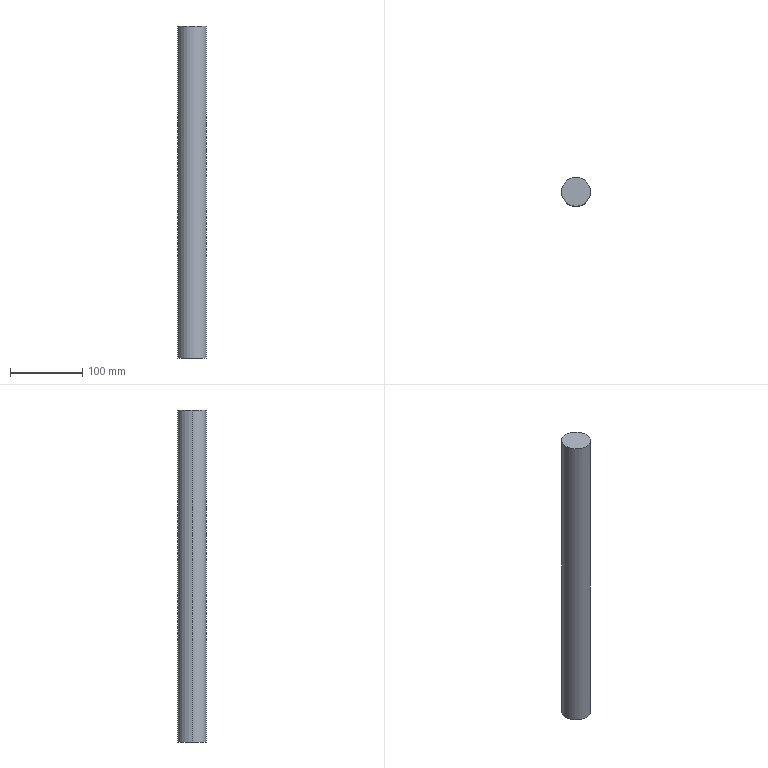Component | SolidWorks | 40Axis-4 | 1 solid | 12 faces | box 40 x 40 x 460 mm | volume 576569 mm3 | cylinder 6 | cone 4 | plane 2 | commonest cylinder face diameters 6.8 x4 40 x2 | material 45#
build123d program:
from build123d import *

# Parameters (mm, degrees)
SKETCH1_R             = 20
BOSS_EXTRUDE1_DEPTH   = 230
M8_TAPPED_HOLE1_D     = 6.8
M8_TAPPED_HOLE1_DEPTH = 19.75
M8_TAPPED_HOLE1_TIP   = 2.043


with BuildPart() as part:
    # Sketch1 → Boss-Extrude1 (new, symmetric)
    with BuildSketch(Plane.XY):
        Circle(SKETCH1_R)
    extrude(amount=BOSS_EXTRUDE1_DEPTH, both=True)

    # M8 Tapped Hole1
    with Locations(Plane(origin=(-10, 0, -230), x_dir=(-1, 0, 0), z_dir=(0, 0, -1))):
        with Locations((0, 0), (-20, 0)):
            Hole(M8_TAPPED_HOLE1_D / 2, depth=M8_TAPPED_HOLE1_DEPTH)
            with Locations((0, 0, -(M8_TAPPED_HOLE1_DEPTH + M8_TAPPED_HOLE1_TIP / 2))):  # 118° drill point
                Cone(0, M8_TAPPED_HOLE1_D / 2, M8_TAPPED_HOLE1_TIP, mode=Mode.SUBTRACT)


solid = part.part

# Placed as in the assembly
solid = solid.moved(Location((-218.215, 103.083, -950.957), (0, 0, 0)))
STEP:
#1=COLOUR_RGB('',0.7922,0.8196,0.9333);
#2=FILL_AREA_STYLE_COLOUR('',#1);
#3=FILL_AREA_STYLE('',(#2));
#4=SURFACE_STYLE_FILL_AREA(#3);
#5=SURFACE_SIDE_STYLE('',(#4));
#6=SURFACE_STYLE_USAGE(.BOTH.,#5);
#7=PRESENTATION_STYLE_ASSIGNMENT((#6));
#8=CARTESIAN_POINT('',(-8.331,4.058,-45.717));
#9=VERTEX_POINT('',#8);
#10=CARTESIAN_POINT('',(-8.064,4.058,-45.717));
#11=VERTEX_POINT('',#10);
#12=CARTESIAN_POINT('',(-8.197,4.058,-45.717));
#13=DIRECTION('',(0.,-0.,-1.));
#14=DIRECTION('',(1.,0.,0.));
#15=AXIS2_PLACEMENT_3D('',#12,#13,#14);
#16=CIRCLE('',#15,0.1339);
#17=EDGE_CURVE('',#9,#11,#16,.T.);
#18=ORIENTED_EDGE('',*,*,#17,.F.);
#19=CARTESIAN_POINT('',(-8.331,4.058,-46.494));
#20=VERTEX_POINT('',#19);
#21=CARTESIAN_POINT('',(-8.331,4.058,-46.494));
#22=DIRECTION('',(0.,-0.,-1.));
#23=VECTOR('',#22,39.37);
#24=LINE('',#21,#23);
#25=EDGE_CURVE('',#9,#20,#24,.T.);
#26=ORIENTED_EDGE('',*,*,#25,.T.);
#27=CARTESIAN_POINT('',(-8.064,4.058,-46.494));
#28=VERTEX_POINT('',#27);
#29=CARTESIAN_POINT('',(-8.197,4.058,-46.494));
#30=DIRECTION('',(0.,-0.,-1.));
#31=DIRECTION('',(1.,0.,0.));
#32=AXIS2_PLACEMENT_3D('',#29,#30,#31);
#33=CIRCLE('',#32,0.1339);
#34=EDGE_CURVE('',#20,#28,#33,.T.);
#35=ORIENTED_EDGE('',*,*,#34,.T.);
#36=CARTESIAN_POINT('',(-8.064,4.058,-46.494));
#37=DIRECTION('',(0.,-0.,-1.));
#38=VECTOR('',#37,39.37);
#39=LINE('',#36,#38);
#40=EDGE_CURVE('',#11,#28,#39,.T.);
#41=ORIENTED_EDGE('',*,*,#40,.F.);
#42=EDGE_LOOP('',(#18,#26,#35,#41));
#43=FACE_OUTER_BOUND('',#42,.T.);
#44=CARTESIAN_POINT('',(-8.197,4.058,-46.494));
#45=DIRECTION('',(0.,-0.,-1.));
#46=DIRECTION('',(1.,0.,0.));
#47=AXIS2_PLACEMENT_3D('',#44,#45,#46);
#48=CYLINDRICAL_SURFACE('',#47,0.1339);
#49=ADVANCED_FACE('',(#43),#48,.F.);
#50=CARTESIAN_POINT('',(-8.197,4.058,-45.636));
#51=VERTEX_POINT('',#50);
#52=CARTESIAN_POINT('',(-8.064,4.058,-45.717));
#53=DIRECTION('',(0.8572,0.,-0.515));
#54=VECTOR('',#53,39.37);
#55=LINE('',#52,#54);
#56=EDGE_CURVE('',#51,#11,#55,.T.);
#57=ORIENTED_EDGE('',*,*,#56,.F.);
#58=CARTESIAN_POINT('',(-8.331,4.058,-45.717));
#59=DIRECTION('',(-0.8572,-0.,-0.515));
#60=VECTOR('',#59,39.37);
#61=LINE('',#58,#60);
#62=EDGE_CURVE('',#51,#9,#61,.T.);
#63=ORIENTED_EDGE('',*,*,#62,.T.);
#64=ORIENTED_EDGE('',*,*,#17,.T.);
#65=EDGE_LOOP('',(#57,#63,#64));
#66=FACE_OUTER_BOUND('',#65,.T.);
#67=CARTESIAN_POINT('',(-8.197,4.058,-45.717));
#68=DIRECTION('',(0.,-0.,-1.));
#69=DIRECTION('',(1.,0.,0.));
#70=AXIS2_PLACEMENT_3D('',#67,#68,#69);
#71=CONICAL_SURFACE('',#70,0.1339,1.03);
#72=ADVANCED_FACE('',(#66),#71,.F.);
#73=CARTESIAN_POINT('',(-9.119,4.058,-45.717));
#74=VERTEX_POINT('',#73);
#75=CARTESIAN_POINT('',(-8.851,4.058,-45.717));
#76=VERTEX_POINT('',#75);
#77=CARTESIAN_POINT('',(-8.985,4.058,-45.717));
#78=DIRECTION('',(0.,-0.,-1.));
#79=DIRECTION('',(1.,0.,0.));
#80=AXIS2_PLACEMENT_3D('',#77,#78,#79);
#81=CIRCLE('',#80,0.1339);
#82=EDGE_CURVE('',#74,#76,#81,.T.);
#83=ORIENTED_EDGE('',*,*,#82,.F.);
#84=CARTESIAN_POINT('',(-9.119,4.058,-46.494));
#85=VERTEX_POINT('',#84);
#86=CARTESIAN_POINT('',(-9.119,4.058,-46.494));
#87=DIRECTION('',(0.,-0.,-1.));
#88=VECTOR('',#87,39.37);
#89=LINE('',#86,#88);
#90=EDGE_CURVE('',#74,#85,#89,.T.);
#91=ORIENTED_EDGE('',*,*,#90,.T.);
#92=CARTESIAN_POINT('',(-8.851,4.058,-46.494));
#93=VERTEX_POINT('',#92);
#94=CARTESIAN_POINT('',(-8.985,4.058,-46.494));
#95=DIRECTION('',(0.,-0.,-1.));
#96=DIRECTION('',(1.,0.,0.));
#97=AXIS2_PLACEMENT_3D('',#94,#95,#96);
#98=CIRCLE('',#97,0.1339);
#99=EDGE_CURVE('',#85,#93,#98,.T.);
#100=ORIENTED_EDGE('',*,*,#99,.T.);
#101=CARTESIAN_POINT('',(-8.851,4.058,-46.494));
#102=DIRECTION('',(0.,-0.,-1.));
#103=VECTOR('',#102,39.37);
#104=LINE('',#101,#103);
#105=EDGE_CURVE('',#76,#93,#104,.T.);
#106=ORIENTED_EDGE('',*,*,#105,.F.);
#107=EDGE_LOOP('',(#83,#91,#100,#106));
#108=FACE_OUTER_BOUND('',#107,.T.);
#109=CARTESIAN_POINT('',(-8.985,4.058,-46.494));
#110=DIRECTION('',(0.,-0.,-1.));
#111=DIRECTION('',(1.,0.,0.));
#112=AXIS2_PLACEMENT_3D('',#109,#110,#111);
#113=CYLINDRICAL_SURFACE('',#112,0.1339);
#114=ADVANCED_FACE('',(#108),#113,.F.);
#115=CARTESIAN_POINT('',(-8.985,4.058,-45.636));
#116=VERTEX_POINT('',#115);
#117=CARTESIAN_POINT('',(-8.851,4.058,-45.717));
#118=DIRECTION('',(0.8572,0.,-0.515));
#119=VECTOR('',#118,39.37);
#120=LINE('',#117,#119);
#121=EDGE_CURVE('',#116,#76,#120,.T.);
#122=ORIENTED_EDGE('',*,*,#121,.F.);
#123=CARTESIAN_POINT('',(-9.119,4.058,-45.717));
#124=DIRECTION('',(-0.8572,-0.,-0.515));
#125=VECTOR('',#124,39.37);
#126=LINE('',#123,#125);
#127=EDGE_CURVE('',#116,#74,#126,.T.);
#128=ORIENTED_EDGE('',*,*,#127,.T.);
#129=ORIENTED_EDGE('',*,*,#82,.T.);
#130=EDGE_LOOP('',(#122,#128,#129));
#131=FACE_OUTER_BOUND('',#130,.T.);
#132=CARTESIAN_POINT('',(-8.985,4.058,-45.717));
#133=DIRECTION('',(0.,-0.,-1.));
#134=DIRECTION('',(1.,0.,0.));
#135=AXIS2_PLACEMENT_3D('',#132,#133,#134);
#136=CONICAL_SURFACE('',#135,0.1339,1.03);
#137=ADVANCED_FACE('',(#131),#136,.F.);
#138=CARTESIAN_POINT('',(-9.379,4.058,-28.384));
#139=VERTEX_POINT('',#138);
#140=CARTESIAN_POINT('',(-7.804,4.058,-28.384));
#141=VERTEX_POINT('',#140);
#142=CARTESIAN_POINT('',(-8.591,4.058,-28.384));
#143=DIRECTION('',(-0.,0.,1.));
#144=DIRECTION('',(-1.,-0.,0.));
#145=AXIS2_PLACEMENT_3D('',#142,#143,#144);
#146=CIRCLE('',#145,0.7874);
#147=EDGE_CURVE('',#139,#141,#146,.T.);
#148=ORIENTED_EDGE('',*,*,#147,.F.);
#149=CARTESIAN_POINT('',(-9.379,4.058,-46.494));
#150=VERTEX_POINT('',#149);
#151=CARTESIAN_POINT('',(-9.379,4.058,-28.384));
#152=DIRECTION('',(0.,-0.,-1.));
#153=VECTOR('',#152,39.37);
#154=LINE('',#151,#153);
#155=EDGE_CURVE('',#139,#150,#154,.T.);
#156=ORIENTED_EDGE('',*,*,#155,.T.);
#157=CARTESIAN_POINT('',(-7.804,4.058,-46.494));
#158=VERTEX_POINT('',#157);
#159=CARTESIAN_POINT('',(-8.591,4.058,-46.494));
#160=DIRECTION('',(-0.,0.,1.));
#161=DIRECTION('',(-1.,-0.,0.));
#162=AXIS2_PLACEMENT_3D('',#159,#160,#161);
#163=CIRCLE('',#162,0.7874);
#164=EDGE_CURVE('',#150,#158,#163,.T.);
#165=ORIENTED_EDGE('',*,*,#164,.T.);
#166=CARTESIAN_POINT('',(-7.804,4.058,-28.384));
#167=DIRECTION('',(0.,-0.,-1.));
#168=VECTOR('',#167,39.37);
#169=LINE('',#166,#168);
#170=EDGE_CURVE('',#141,#158,#169,.T.);
#171=ORIENTED_EDGE('',*,*,#170,.F.);
#172=EDGE_LOOP('',(#148,#156,#165,#171));
#173=FACE_OUTER_BOUND('',#172,.T.);
#174=CARTESIAN_POINT('',(-8.591,4.058,-28.384));
#175=DIRECTION('',(0.,-0.,-1.));
#176=DIRECTION('',(1.,0.,0.));
#177=AXIS2_PLACEMENT_3D('',#174,#175,#176);
#178=CYLINDRICAL_SURFACE('',#177,0.7874);
#179=ADVANCED_FACE('',(#173),#178,.T.);
#180=ORIENTED_EDGE('',*,*,#155,.F.);
#181=CARTESIAN_POINT('',(-8.591,4.058,-28.384));
#182=DIRECTION('',(-0.,0.,1.));
#183=DIRECTION('',(-1.,-0.,0.));
#184=AXIS2_PLACEMENT_3D('',#181,#182,#183);
#185=CIRCLE('',#184,0.7874);
#186=EDGE_CURVE('',#141,#139,#185,.T.);
#187=ORIENTED_EDGE('',*,*,#186,.F.);
#188=ORIENTED_EDGE('',*,*,#170,.T.);
#189=CARTESIAN_POINT('',(-8.591,4.058,-46.494));
#190=DIRECTION('',(-0.,0.,1.));
#191=DIRECTION('',(-1.,-0.,0.));
#192=AXIS2_PLACEMENT_3D('',#189,#190,#191);
#193=CIRCLE('',#192,0.7874);
#194=EDGE_CURVE('',#158,#150,#193,.T.);
#195=ORIENTED_EDGE('',*,*,#194,.T.);
#196=EDGE_LOOP('',(#180,#187,#188,#195));
#197=FACE_OUTER_BOUND('',#196,.T.);
#198=CARTESIAN_POINT('',(-8.591,4.058,-28.384));
#199=DIRECTION('',(0.,-0.,-1.));
#200=DIRECTION('',(1.,0.,0.));
#201=AXIS2_PLACEMENT_3D('',#198,#199,#200);
#202=CYLINDRICAL_SURFACE('',#201,0.7874);
#203=ADVANCED_FACE('',(#197),#202,.T.);
#204=ORIENTED_EDGE('',*,*,#186,.T.);
#205=ORIENTED_EDGE('',*,*,#147,.T.);
#206=EDGE_LOOP('',(#204,#205));
#207=FACE_OUTER_BOUND('',#206,.T.);
#208=CARTESIAN_POINT('',(-8.591,4.058,-28.384));
#209=DIRECTION('',(-0.,0.,1.));
#210=DIRECTION('',(-1.,-0.,-0.));
#211=AXIS2_PLACEMENT_3D('',#208,#209,#210);
#212=PLANE('',#211);
#213=ADVANCED_FACE('',(#207),#212,.T.);
#214=CARTESIAN_POINT('',(-8.197,4.058,-46.494));
#215=DIRECTION('',(0.,-0.,-1.));
#216=DIRECTION('',(1.,0.,0.));
#217=AXIS2_PLACEMENT_3D('',#214,#215,#216);
#218=CIRCLE('',#217,0.1339);
#219=EDGE_CURVE('',#28,#20,#218,.T.);
#220=ORIENTED_EDGE('',*,*,#219,.F.);
#221=ORIENTED_EDGE('',*,*,#34,.F.);
#222=EDGE_LOOP('',(#220,#221));
#223=FACE_BOUND('',#222,.T.);
#224=CARTESIAN_POINT('',(-8.985,4.058,-46.494));
#225=DIRECTION('',(0.,-0.,-1.));
#226=DIRECTION('',(1.,0.,0.));
#227=AXIS2_PLACEMENT_3D('',#224,#225,#226);
#228=CIRCLE('',#227,0.1339);
#229=EDGE_CURVE('',#93,#85,#228,.T.);
#230=ORIENTED_EDGE('',*,*,#229,.F.);
#231=ORIENTED_EDGE('',*,*,#99,.F.);
#232=EDGE_LOOP('',(#230,#231));
#233=FACE_BOUND('',#232,.T.);
#234=ORIENTED_EDGE('',*,*,#194,.F.);
#235=ORIENTED_EDGE('',*,*,#164,.F.);
#236=EDGE_LOOP('',(#234,#235));
#237=FACE_OUTER_BOUND('',#236,.T.);
#238=CARTESIAN_POINT('',(-8.591,4.058,-46.494));
#239=DIRECTION('',(-0.,0.,1.));
#240=DIRECTION('',(-1.,-0.,-0.));
#241=AXIS2_PLACEMENT_3D('',#238,#239,#240);
#242=PLANE('',#241);
#243=ADVANCED_FACE('',(#223,#233,#237),#242,.F.);
#244=ORIENTED_EDGE('',*,*,#127,.F.);
#245=ORIENTED_EDGE('',*,*,#121,.T.);
#246=CARTESIAN_POINT('',(-8.985,4.058,-45.717));
#247=DIRECTION('',(0.,-0.,-1.));
#248=DIRECTION('',(1.,0.,0.));
#249=AXIS2_PLACEMENT_3D('',#246,#247,#248);
#250=CIRCLE('',#249,0.1339);
#251=EDGE_CURVE('',#76,#74,#250,.T.);
#252=ORIENTED_EDGE('',*,*,#251,.T.);
#253=EDGE_LOOP('',(#244,#245,#252));
#254=FACE_OUTER_BOUND('',#253,.T.);
#255=CARTESIAN_POINT('',(-8.985,4.058,-45.717));
#256=DIRECTION('',(0.,-0.,-1.));
#257=DIRECTION('',(1.,0.,0.));
#258=AXIS2_PLACEMENT_3D('',#255,#256,#257);
#259=CONICAL_SURFACE('',#258,0.1339,1.03);
#260=ADVANCED_FACE('',(#254),#259,.F.);
#261=ORIENTED_EDGE('',*,*,#90,.F.);
#262=ORIENTED_EDGE('',*,*,#251,.F.);
#263=ORIENTED_EDGE('',*,*,#105,.T.);
#264=ORIENTED_EDGE('',*,*,#229,.T.);
#265=EDGE_LOOP('',(#261,#262,#263,#264));
#266=FACE_OUTER_BOUND('',#265,.T.);
#267=CARTESIAN_POINT('',(-8.985,4.058,-46.494));
#268=DIRECTION('',(0.,-0.,-1.));
#269=DIRECTION('',(1.,0.,0.));
#270=AXIS2_PLACEMENT_3D('',#267,#268,#269);
#271=CYLINDRICAL_SURFACE('',#270,0.1339);
#272=ADVANCED_FACE('',(#266),#271,.F.);
#273=ORIENTED_EDGE('',*,*,#62,.F.);
#274=ORIENTED_EDGE('',*,*,#56,.T.);
#275=CARTESIAN_POINT('',(-8.197,4.058,-45.717));
#276=DIRECTION('',(0.,-0.,-1.));
#277=DIRECTION('',(1.,0.,0.));
#278=AXIS2_PLACEMENT_3D('',#275,#276,#277);
#279=CIRCLE('',#278,0.1339);
#280=EDGE_CURVE('',#11,#9,#279,.T.);
#281=ORIENTED_EDGE('',*,*,#280,.T.);
#282=EDGE_LOOP('',(#273,#274,#281));
#283=FACE_OUTER_BOUND('',#282,.T.);
#284=CARTESIAN_POINT('',(-8.197,4.058,-45.717));
#285=DIRECTION('',(0.,-0.,-1.));
#286=DIRECTION('',(1.,0.,0.));
#287=AXIS2_PLACEMENT_3D('',#284,#285,#286);
#288=CONICAL_SURFACE('',#287,0.1339,1.03);
#289=ADVANCED_FACE('',(#283),#288,.F.);
#290=ORIENTED_EDGE('',*,*,#25,.F.);
#291=ORIENTED_EDGE('',*,*,#280,.F.);
#292=ORIENTED_EDGE('',*,*,#40,.T.);
#293=ORIENTED_EDGE('',*,*,#219,.T.);
#294=EDGE_LOOP('',(#290,#291,#292,#293));
#295=FACE_OUTER_BOUND('',#294,.T.);
#296=CARTESIAN_POINT('',(-8.197,4.058,-46.494));
#297=DIRECTION('',(0.,-0.,-1.));
#298=DIRECTION('',(1.,0.,0.));
#299=AXIS2_PLACEMENT_3D('',#296,#297,#298);
#300=CYLINDRICAL_SURFACE('',#299,0.1339);
#301=ADVANCED_FACE('',(#295),#300,.F.);
#302=CLOSED_SHELL('',(#49,#72,#114,#137,#179,#203,#213,#243,#260,#272,#289,#301));
#303=MANIFOLD_SOLID_BREP('',#302);
#304=STYLED_ITEM('',(#7),#303);
#305=PRESENTATION_LAYER_ASSIGNMENT('','',(#304));
#306=CARTESIAN_POINT('',(0.,0.,0.));
#307=DIRECTION('',(0.,0.,1.));
#308=DIRECTION('',(1.,0.,0.));
#309=AXIS2_PLACEMENT_3D('',#306,#307,#308);
#310=(LENGTH_UNIT()NAMED_UNIT(*)SI_UNIT($,.METRE.));
#311=LENGTH_MEASURE_WITH_UNIT(LENGTH_MEASURE(0.0254),#310);
#312=DIMENSIONAL_EXPONENTS(1.,0.,0.,0.,0.,0.,0.);
#313=(CONVERSION_BASED_UNIT('',#311)LENGTH_UNIT()NAMED_UNIT(#312));
#314=UNCERTAINTY_MEASURE_WITH_UNIT(LENGTH_MEASURE(0.00001),#313,'','');
#315=(NAMED_UNIT(*)PLANE_ANGLE_UNIT()SI_UNIT($,.RADIAN.));
#316=(NAMED_UNIT(*)SI_UNIT($,.STERADIAN.)SOLID_ANGLE_UNIT());
#317=(GEOMETRIC_REPRESENTATION_CONTEXT(3)GLOBAL_UNCERTAINTY_ASSIGNED_CONTEXT((#314))GLOBAL_UNIT_ASSIGNED_CONTEXT((#313,#315,#316))REPRESENTATION_CONTEXT('',''));
#318=ADVANCED_BREP_SHAPE_REPRESENTATION('',(#303,#309),#317);
#319=(LENGTH_UNIT()NAMED_UNIT(*)SI_UNIT($,.METRE.));
#320=LENGTH_MEASURE_WITH_UNIT(LENGTH_MEASURE(0.0254),#319);
#321=DIMENSIONAL_EXPONENTS(1.,0.,0.,0.,0.,0.,0.);
#322=(CONVERSION_BASED_UNIT('',#320)LENGTH_UNIT()NAMED_UNIT(#321));
#323=UNCERTAINTY_MEASURE_WITH_UNIT(LENGTH_MEASURE(0.00001),#322,'','');
#324=(NAMED_UNIT(*)PLANE_ANGLE_UNIT()SI_UNIT($,.RADIAN.));
#325=(NAMED_UNIT(*)SI_UNIT($,.STERADIAN.)SOLID_ANGLE_UNIT());
#326=(GEOMETRIC_REPRESENTATION_CONTEXT(3)GLOBAL_UNCERTAINTY_ASSIGNED_CONTEXT((#323))GLOBAL_UNIT_ASSIGNED_CONTEXT((#322,#324,#325))REPRESENTATION_CONTEXT('',''));
#327=MECHANICAL_DESIGN_GEOMETRIC_PRESENTATION_REPRESENTATION('',(#304),#326);